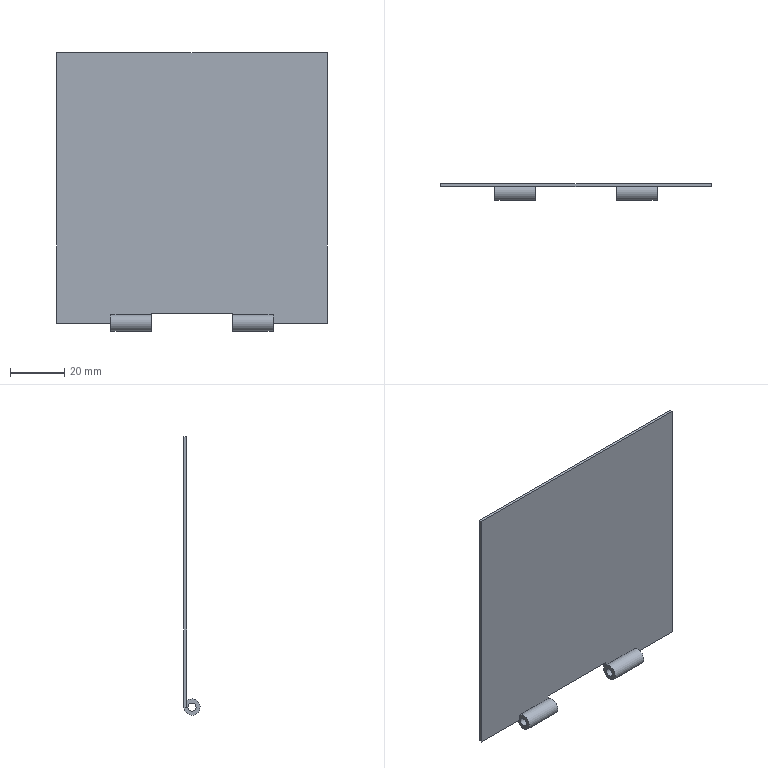Component | NX | PART_7 | 1 solid | 16 faces | box 100 x 6 x 103 mm | volume 10485 mm3 | plane 12 | cylinder 4 | commonest cylinder face diameters 6 x2 3 x2
STEP:
#1=CARTESIAN_POINT('',(0.,0.,0.));
#2=DIRECTION('',(0.,0.,1.));
#3=DIRECTION('',(1.,0.,0.));
#4=AXIS2_PLACEMENT_3D('',#1,#2,#3);
#5=CARTESIAN_POINT('',(-30.,28.,-0.));
#6=VERTEX_POINT('',#5);
#7=CARTESIAN_POINT('',(-30.,29.,-0.));
#8=VERTEX_POINT('',#7);
#9=CARTESIAN_POINT('',(-30.,29.,-0.));
#10=DIRECTION('',(0.,1.,0.));
#11=VECTOR('',#10,1.);
#12=LINE('',#9,#11);
#13=CARTESIAN_POINT('',(50.,29.,-0.));
#14=DIRECTION('',(0.,-0.,1.));
#15=DIRECTION('',(0.,-1.,-0.));
#16=AXIS2_PLACEMENT_3D('',#13,#14,#15);
#17=PLANE('',#16);
#18=CARTESIAN_POINT('',(0.,-80.));
#19=DIRECTION('',(-1.,0.));
#20=VECTOR('',#19,1.);
#21=LINE('',#18,#20);
#22=(GEOMETRIC_REPRESENTATION_CONTEXT(2)PARAMETRIC_REPRESENTATION_CONTEXT()REPRESENTATION_CONTEXT('',''));
#23=DEFINITIONAL_REPRESENTATION('',(#21),#22);
#24=PCURVE('',#17,#23);
#25=CARTESIAN_POINT('',(-30.,26.,-0.));
#26=DIRECTION('',(1.,0.,0.));
#27=DIRECTION('',(0.,0.,1.));
#28=AXIS2_PLACEMENT_3D('',#25,#26,#27);
#29=PLANE('',#28);
#30=CARTESIAN_POINT('',(0.,-3.));
#31=DIRECTION('',(0.,-1.));
#32=VECTOR('',#31,1.);
#33=LINE('',#30,#32);
#34=(GEOMETRIC_REPRESENTATION_CONTEXT(2)PARAMETRIC_REPRESENTATION_CONTEXT()REPRESENTATION_CONTEXT('',''));
#35=DEFINITIONAL_REPRESENTATION('',(#33),#34);
#36=PCURVE('',#29,#35);
#37=SURFACE_CURVE('',#12,(#24,#36),.PCURVE_S1.);
#38=EDGE_CURVE('',#6,#8,#37,.T.);
#39=ORIENTED_EDGE('',*,*,#38,.F.);
#40=CARTESIAN_POINT('',(-50.,28.,-0.));
#41=VERTEX_POINT('',#40);
#42=CARTESIAN_POINT('',(50.,28.,-0.));
#43=DIRECTION('',(-1.,0.,0.));
#44=VECTOR('',#43,1.);
#45=LINE('',#42,#44);
#46=CARTESIAN_POINT('',(1.,0.));
#47=DIRECTION('',(0.,-1.));
#48=VECTOR('',#47,1.);
#49=LINE('',#46,#48);
#50=(GEOMETRIC_REPRESENTATION_CONTEXT(2)PARAMETRIC_REPRESENTATION_CONTEXT()REPRESENTATION_CONTEXT('',''));
#51=DEFINITIONAL_REPRESENTATION('',(#49),#50);
#52=PCURVE('',#17,#51);
#53=CARTESIAN_POINT('',(50.,28.,100.));
#54=DIRECTION('',(0.,1.,0.));
#55=DIRECTION('',(0.,-0.,1.));
#56=AXIS2_PLACEMENT_3D('',#53,#54,#55);
#57=PLANE('',#56);
#58=CARTESIAN_POINT('',(-100.,0.));
#59=DIRECTION('',(0.,-1.));
#60=VECTOR('',#59,1.);
#61=LINE('',#58,#60);
#62=(GEOMETRIC_REPRESENTATION_CONTEXT(2)PARAMETRIC_REPRESENTATION_CONTEXT()REPRESENTATION_CONTEXT('',''));
#63=DEFINITIONAL_REPRESENTATION('',(#61),#62);
#64=PCURVE('',#57,#63);
#65=SURFACE_CURVE('',#45,(#52,#64),.PCURVE_S1.);
#66=EDGE_CURVE('',#6,#41,#65,.T.);
#67=ORIENTED_EDGE('',*,*,#66,.T.);
#68=CARTESIAN_POINT('',(-50.,29.,-0.));
#69=VERTEX_POINT('',#68);
#70=CARTESIAN_POINT('',(-50.,31.,-0.));
#71=DIRECTION('',(0.,1.,0.));
#72=VECTOR('',#71,1.);
#73=LINE('',#70,#72);
#74=CARTESIAN_POINT('',(-2.,-100.));
#75=DIRECTION('',(-1.,0.));
#76=VECTOR('',#75,1.);
#77=LINE('',#74,#76);
#78=(GEOMETRIC_REPRESENTATION_CONTEXT(2)PARAMETRIC_REPRESENTATION_CONTEXT()REPRESENTATION_CONTEXT('',''));
#79=DEFINITIONAL_REPRESENTATION('',(#77),#78);
#80=PCURVE('',#17,#79);
#81=CARTESIAN_POINT('',(-50.,31.,100.));
#82=DIRECTION('',(-1.,0.,0.));
#83=DIRECTION('',(0.,0.,-1.));
#84=AXIS2_PLACEMENT_3D('',#81,#82,#83);
#85=PLANE('',#84);
#86=CARTESIAN_POINT('',(100.,0.));
#87=DIRECTION('',(-0.,-1.));
#88=VECTOR('',#87,1.);
#89=LINE('',#86,#88);
#90=(GEOMETRIC_REPRESENTATION_CONTEXT(2)PARAMETRIC_REPRESENTATION_CONTEXT()REPRESENTATION_CONTEXT('',''));
#91=DEFINITIONAL_REPRESENTATION('',(#89),#90);
#92=PCURVE('',#85,#91);
#93=SURFACE_CURVE('',#73,(#80,#92),.PCURVE_S1.);
#94=EDGE_CURVE('',#41,#69,#93,.T.);
#95=ORIENTED_EDGE('',*,*,#94,.T.);
#96=CARTESIAN_POINT('',(50.,29.,-0.));
#97=DIRECTION('',(-1.,0.,0.));
#98=VECTOR('',#97,1.);
#99=LINE('',#96,#98);
#100=CARTESIAN_POINT('',(0.,0.));
#101=DIRECTION('',(0.,-1.));
#102=VECTOR('',#101,1.);
#103=LINE('',#100,#102);
#104=(GEOMETRIC_REPRESENTATION_CONTEXT(2)PARAMETRIC_REPRESENTATION_CONTEXT()REPRESENTATION_CONTEXT('',''));
#105=DEFINITIONAL_REPRESENTATION('',(#103),#104);
#106=PCURVE('',#17,#105);
#107=CARTESIAN_POINT('',(50.,29.,-0.));
#108=DIRECTION('',(0.,-1.,-0.));
#109=DIRECTION('',(0.,0.,-1.));
#110=AXIS2_PLACEMENT_3D('',#107,#108,#109);
#111=PLANE('',#110);
#112=CARTESIAN_POINT('',(-0.,0.));
#113=DIRECTION('',(0.,-1.));
#114=VECTOR('',#113,1.);
#115=LINE('',#112,#114);
#116=(GEOMETRIC_REPRESENTATION_CONTEXT(2)PARAMETRIC_REPRESENTATION_CONTEXT()REPRESENTATION_CONTEXT('',''));
#117=DEFINITIONAL_REPRESENTATION('',(#115),#116);
#118=PCURVE('',#111,#117);
#119=SURFACE_CURVE('',#99,(#106,#118),.PCURVE_S1.);
#120=EDGE_CURVE('',#8,#69,#119,.T.);
#121=ORIENTED_EDGE('',*,*,#120,.F.);
#122=EDGE_LOOP('',(#39,#67,#95,#121));
#123=FACE_BOUND('',#122,.T.);
#124=ADVANCED_FACE('',(#123),#17,.F.);
#125=CARTESIAN_POINT('',(-30.,28.,2.236));
#126=VERTEX_POINT('',#125);
#127=CARTESIAN_POINT('',(-15.,28.,2.236));
#128=VERTEX_POINT('',#127);
#129=CARTESIAN_POINT('',(-30.,28.,2.236));
#130=DIRECTION('',(1.,0.,0.));
#131=VECTOR('',#130,1.);
#132=LINE('',#129,#131);
#133=CARTESIAN_POINT('',(-97.764,-80.));
#134=DIRECTION('',(0.,1.));
#135=VECTOR('',#134,1.);
#136=LINE('',#133,#135);
#137=(GEOMETRIC_REPRESENTATION_CONTEXT(2)PARAMETRIC_REPRESENTATION_CONTEXT()REPRESENTATION_CONTEXT('',''));
#138=DEFINITIONAL_REPRESENTATION('',(#136),#137);
#139=PCURVE('',#57,#138);
#140=CARTESIAN_POINT('',(-30.,26.,-0.));
#141=DIRECTION('',(1.,0.,0.));
#142=DIRECTION('',(0.,0.,1.));
#143=AXIS2_PLACEMENT_3D('',#140,#141,#142);
#144=CYLINDRICAL_SURFACE('',#143,3.);
#145=CARTESIAN_POINT('',(-0.7297,0.));
#146=DIRECTION('',(0.,1.));
#147=VECTOR('',#146,1.);
#148=LINE('',#145,#147);
#149=(GEOMETRIC_REPRESENTATION_CONTEXT(2)PARAMETRIC_REPRESENTATION_CONTEXT()REPRESENTATION_CONTEXT('',''));
#150=DEFINITIONAL_REPRESENTATION('',(#148),#149);
#151=PCURVE('',#144,#150);
#152=SURFACE_CURVE('',#132,(#139,#151),.PCURVE_S1.);
#153=EDGE_CURVE('',#126,#128,#152,.T.);
#154=ORIENTED_EDGE('',*,*,#153,.T.);
#155=CARTESIAN_POINT('',(-15.,28.,3.5));
#156=VERTEX_POINT('',#155);
#157=CARTESIAN_POINT('',(-15.,28.,100.));
#158=DIRECTION('',(0.,-0.,1.));
#159=VECTOR('',#158,1.);
#160=LINE('',#157,#159);
#161=CARTESIAN_POINT('',(0.,-65.));
#162=DIRECTION('',(1.,0.));
#163=VECTOR('',#162,1.);
#164=LINE('',#161,#163);
#165=(GEOMETRIC_REPRESENTATION_CONTEXT(2)PARAMETRIC_REPRESENTATION_CONTEXT()REPRESENTATION_CONTEXT('',''));
#166=DEFINITIONAL_REPRESENTATION('',(#164),#165);
#167=PCURVE('',#57,#166);
#168=CARTESIAN_POINT('',(-15.,26.,-0.));
#169=DIRECTION('',(1.,0.,0.));
#170=DIRECTION('',(0.,0.,1.));
#171=AXIS2_PLACEMENT_3D('',#168,#169,#170);
#172=PLANE('',#171);
#173=CARTESIAN_POINT('',(100.,-2.));
#174=DIRECTION('',(1.,0.));
#175=VECTOR('',#174,1.);
#176=LINE('',#173,#175);
#177=(GEOMETRIC_REPRESENTATION_CONTEXT(2)PARAMETRIC_REPRESENTATION_CONTEXT()REPRESENTATION_CONTEXT('',''));
#178=DEFINITIONAL_REPRESENTATION('',(#176),#177);
#179=PCURVE('',#172,#178);
#180=SURFACE_CURVE('',#160,(#167,#179),.PCURVE_S1.);
#181=EDGE_CURVE('',#128,#156,#180,.T.);
#182=ORIENTED_EDGE('',*,*,#181,.T.);
#183=CARTESIAN_POINT('',(15.,28.,3.5));
#184=VERTEX_POINT('',#183);
#185=CARTESIAN_POINT('',(50.,28.,3.5));
#186=DIRECTION('',(1.,0.,0.));
#187=VECTOR('',#186,1.);
#188=LINE('',#185,#187);
#189=CARTESIAN_POINT('',(-96.5,0.));
#190=DIRECTION('',(0.,1.));
#191=VECTOR('',#190,1.);
#192=LINE('',#189,#191);
#193=(GEOMETRIC_REPRESENTATION_CONTEXT(2)PARAMETRIC_REPRESENTATION_CONTEXT()REPRESENTATION_CONTEXT('',''));
#194=DEFINITIONAL_REPRESENTATION('',(#192),#193);
#195=PCURVE('',#57,#194);
#196=CARTESIAN_POINT('',(0.,28.5,3.5));
#197=DIRECTION('',(0.,0.,1.));
#198=DIRECTION('',(-1.,0.,0.));
#199=AXIS2_PLACEMENT_3D('',#196,#197,#198);
#200=PLANE('',#199);
#201=CARTESIAN_POINT('',(-50.,0.5));
#202=DIRECTION('',(-1.,0.));
#203=VECTOR('',#202,1.);
#204=LINE('',#201,#203);
#205=(GEOMETRIC_REPRESENTATION_CONTEXT(2)PARAMETRIC_REPRESENTATION_CONTEXT()REPRESENTATION_CONTEXT('',''));
#206=DEFINITIONAL_REPRESENTATION('',(#204),#205);
#207=PCURVE('',#200,#206);
#208=SURFACE_CURVE('',#188,(#195,#207),.PCURVE_S1.);
#209=EDGE_CURVE('',#156,#184,#208,.T.);
#210=ORIENTED_EDGE('',*,*,#209,.T.);
#211=CARTESIAN_POINT('',(15.,28.,2.236));
#212=VERTEX_POINT('',#211);
#213=CARTESIAN_POINT('',(15.,28.,100.));
#214=DIRECTION('',(0.,-0.,1.));
#215=VECTOR('',#214,1.);
#216=LINE('',#213,#215);
#217=CARTESIAN_POINT('',(0.,-35.));
#218=DIRECTION('',(1.,0.));
#219=VECTOR('',#218,1.);
#220=LINE('',#217,#219);
#221=(GEOMETRIC_REPRESENTATION_CONTEXT(2)PARAMETRIC_REPRESENTATION_CONTEXT()REPRESENTATION_CONTEXT('',''));
#222=DEFINITIONAL_REPRESENTATION('',(#220),#221);
#223=PCURVE('',#57,#222);
#224=CARTESIAN_POINT('',(15.,26.,-0.));
#225=DIRECTION('',(1.,0.,0.));
#226=DIRECTION('',(0.,0.,1.));
#227=AXIS2_PLACEMENT_3D('',#224,#225,#226);
#228=PLANE('',#227);
#229=CARTESIAN_POINT('',(100.,-2.));
#230=DIRECTION('',(1.,0.));
#231=VECTOR('',#230,1.);
#232=LINE('',#229,#231);
#233=(GEOMETRIC_REPRESENTATION_CONTEXT(2)PARAMETRIC_REPRESENTATION_CONTEXT()REPRESENTATION_CONTEXT('',''));
#234=DEFINITIONAL_REPRESENTATION('',(#232),#233);
#235=PCURVE('',#228,#234);
#236=SURFACE_CURVE('',#216,(#223,#235),.PCURVE_S1.);
#237=EDGE_CURVE('',#212,#184,#236,.T.);
#238=ORIENTED_EDGE('',*,*,#237,.F.);
#239=CARTESIAN_POINT('',(30.,28.,2.236));
#240=VERTEX_POINT('',#239);
#241=CARTESIAN_POINT('',(30.,28.,2.236));
#242=DIRECTION('',(-1.,0.,0.));
#243=VECTOR('',#242,1.);
#244=LINE('',#241,#243);
#245=CARTESIAN_POINT('',(-97.764,-20.));
#246=DIRECTION('',(0.,-1.));
#247=VECTOR('',#246,1.);
#248=LINE('',#245,#247);
#249=(GEOMETRIC_REPRESENTATION_CONTEXT(2)PARAMETRIC_REPRESENTATION_CONTEXT()REPRESENTATION_CONTEXT('',''));
#250=DEFINITIONAL_REPRESENTATION('',(#248),#249);
#251=PCURVE('',#57,#250);
#252=CARTESIAN_POINT('',(30.,26.,-0.));
#253=DIRECTION('',(-1.,0.,0.));
#254=DIRECTION('',(0.,0.,-1.));
#255=AXIS2_PLACEMENT_3D('',#252,#253,#254);
#256=CYLINDRICAL_SURFACE('',#255,3.);
#257=CARTESIAN_POINT('',(3.871,0.));
#258=DIRECTION('',(0.,1.));
#259=VECTOR('',#258,1.);
#260=LINE('',#257,#259);
#261=(GEOMETRIC_REPRESENTATION_CONTEXT(2)PARAMETRIC_REPRESENTATION_CONTEXT()REPRESENTATION_CONTEXT('',''));
#262=DEFINITIONAL_REPRESENTATION('',(#260),#261);
#263=PCURVE('',#256,#262);
#264=SURFACE_CURVE('',#244,(#251,#263),.PCURVE_S1.);
#265=EDGE_CURVE('',#240,#212,#264,.T.);
#266=ORIENTED_EDGE('',*,*,#265,.F.);
#267=CARTESIAN_POINT('',(30.,28.,-0.));
#268=VERTEX_POINT('',#267);
#269=CARTESIAN_POINT('',(30.,28.,100.));
#270=DIRECTION('',(0.,0.,-1.));
#271=VECTOR('',#270,1.);
#272=LINE('',#269,#271);
#273=CARTESIAN_POINT('',(0.,-20.));
#274=DIRECTION('',(-1.,0.));
#275=VECTOR('',#274,1.);
#276=LINE('',#273,#275);
#277=(GEOMETRIC_REPRESENTATION_CONTEXT(2)PARAMETRIC_REPRESENTATION_CONTEXT()REPRESENTATION_CONTEXT('',''));
#278=DEFINITIONAL_REPRESENTATION('',(#276),#277);
#279=PCURVE('',#57,#278);
#280=CARTESIAN_POINT('',(30.,26.,-0.));
#281=DIRECTION('',(1.,0.,0.));
#282=DIRECTION('',(0.,0.,1.));
#283=AXIS2_PLACEMENT_3D('',#280,#281,#282);
#284=PLANE('',#283);
#285=CARTESIAN_POINT('',(100.,-2.));
#286=DIRECTION('',(-1.,-0.));
#287=VECTOR('',#286,1.);
#288=LINE('',#285,#287);
#289=(GEOMETRIC_REPRESENTATION_CONTEXT(2)PARAMETRIC_REPRESENTATION_CONTEXT()REPRESENTATION_CONTEXT('',''));
#290=DEFINITIONAL_REPRESENTATION('',(#288),#289);
#291=PCURVE('',#284,#290);
#292=SURFACE_CURVE('',#272,(#279,#291),.PCURVE_S1.);
#293=EDGE_CURVE('',#240,#268,#292,.T.);
#294=ORIENTED_EDGE('',*,*,#293,.T.);
#295=CARTESIAN_POINT('',(50.,28.,-0.));
#296=VERTEX_POINT('',#295);
#297=CARTESIAN_POINT('',(50.,28.,-0.));
#298=DIRECTION('',(-1.,0.,0.));
#299=VECTOR('',#298,1.);
#300=LINE('',#297,#299);
#301=CARTESIAN_POINT('',(-100.,0.));
#302=DIRECTION('',(0.,-1.));
#303=VECTOR('',#302,1.);
#304=LINE('',#301,#303);
#305=(GEOMETRIC_REPRESENTATION_CONTEXT(2)PARAMETRIC_REPRESENTATION_CONTEXT()REPRESENTATION_CONTEXT('',''));
#306=DEFINITIONAL_REPRESENTATION('',(#304),#305);
#307=PCURVE('',#57,#306);
#308=CARTESIAN_POINT('',(50.,29.,-0.));
#309=DIRECTION('',(0.,-0.,1.));
#310=DIRECTION('',(0.,-1.,-0.));
#311=AXIS2_PLACEMENT_3D('',#308,#309,#310);
#312=PLANE('',#311);
#313=CARTESIAN_POINT('',(1.,0.));
#314=DIRECTION('',(0.,-1.));
#315=VECTOR('',#314,1.);
#316=LINE('',#313,#315);
#317=(GEOMETRIC_REPRESENTATION_CONTEXT(2)PARAMETRIC_REPRESENTATION_CONTEXT()REPRESENTATION_CONTEXT('',''));
#318=DEFINITIONAL_REPRESENTATION('',(#316),#317);
#319=PCURVE('',#312,#318);
#320=SURFACE_CURVE('',#300,(#307,#319),.PCURVE_S1.);
#321=EDGE_CURVE('',#296,#268,#320,.T.);
#322=ORIENTED_EDGE('',*,*,#321,.F.);
#323=CARTESIAN_POINT('',(50.,28.,100.));
#324=VERTEX_POINT('',#323);
#325=CARTESIAN_POINT('',(50.,28.,100.));
#326=DIRECTION('',(0.,0.,-1.));
#327=VECTOR('',#326,1.);
#328=LINE('',#325,#327);
#329=CARTESIAN_POINT('',(0.,0.));
#330=DIRECTION('',(-1.,0.));
#331=VECTOR('',#330,1.);
#332=LINE('',#329,#331);
#333=(GEOMETRIC_REPRESENTATION_CONTEXT(2)PARAMETRIC_REPRESENTATION_CONTEXT()REPRESENTATION_CONTEXT('',''));
#334=DEFINITIONAL_REPRESENTATION('',(#332),#333);
#335=PCURVE('',#57,#334);
#336=CARTESIAN_POINT('',(50.,31.,100.));
#337=DIRECTION('',(-1.,0.,0.));
#338=DIRECTION('',(0.,0.,-1.));
#339=AXIS2_PLACEMENT_3D('',#336,#337,#338);
#340=PLANE('',#339);
#341=CARTESIAN_POINT('',(0.,3.));
#342=DIRECTION('',(1.,-0.));
#343=VECTOR('',#342,1.);
#344=LINE('',#341,#343);
#345=(GEOMETRIC_REPRESENTATION_CONTEXT(2)PARAMETRIC_REPRESENTATION_CONTEXT()REPRESENTATION_CONTEXT('',''));
#346=DEFINITIONAL_REPRESENTATION('',(#344),#345);
#347=PCURVE('',#340,#346);
#348=SURFACE_CURVE('',#328,(#335,#347),.PCURVE_S1.);
#349=EDGE_CURVE('',#324,#296,#348,.T.);
#350=ORIENTED_EDGE('',*,*,#349,.F.);
#351=CARTESIAN_POINT('',(-50.,28.,100.));
#352=VERTEX_POINT('',#351);
#353=CARTESIAN_POINT('',(50.,28.,100.));
#354=DIRECTION('',(-1.,0.,0.));
#355=VECTOR('',#354,1.);
#356=LINE('',#353,#355);
#357=CARTESIAN_POINT('',(0.,0.));
#358=DIRECTION('',(0.,-1.));
#359=VECTOR('',#358,1.);
#360=LINE('',#357,#359);
#361=(GEOMETRIC_REPRESENTATION_CONTEXT(2)PARAMETRIC_REPRESENTATION_CONTEXT()REPRESENTATION_CONTEXT('',''));
#362=DEFINITIONAL_REPRESENTATION('',(#360),#361);
#363=PCURVE('',#57,#362);
#364=CARTESIAN_POINT('',(0.,31.,100.));
#365=DIRECTION('',(0.,0.,-1.));
#366=DIRECTION('',(0.,-1.,0.));
#367=AXIS2_PLACEMENT_3D('',#364,#365,#366);
#368=PLANE('',#367);
#369=CARTESIAN_POINT('',(3.,-50.));
#370=DIRECTION('',(0.,1.));
#371=VECTOR('',#370,1.);
#372=LINE('',#369,#371);
#373=(GEOMETRIC_REPRESENTATION_CONTEXT(2)PARAMETRIC_REPRESENTATION_CONTEXT()REPRESENTATION_CONTEXT('',''));
#374=DEFINITIONAL_REPRESENTATION('',(#372),#373);
#375=PCURVE('',#368,#374);
#376=SURFACE_CURVE('',#356,(#363,#375),.PCURVE_S1.);
#377=EDGE_CURVE('',#324,#352,#376,.T.);
#378=ORIENTED_EDGE('',*,*,#377,.T.);
#379=CARTESIAN_POINT('',(-50.,28.,100.));
#380=DIRECTION('',(0.,0.,-1.));
#381=VECTOR('',#380,1.);
#382=LINE('',#379,#381);
#383=CARTESIAN_POINT('',(0.,-100.));
#384=DIRECTION('',(-1.,0.));
#385=VECTOR('',#384,1.);
#386=LINE('',#383,#385);
#387=(GEOMETRIC_REPRESENTATION_CONTEXT(2)PARAMETRIC_REPRESENTATION_CONTEXT()REPRESENTATION_CONTEXT('',''));
#388=DEFINITIONAL_REPRESENTATION('',(#386),#387);
#389=PCURVE('',#57,#388);
#390=CARTESIAN_POINT('',(0.,3.));
#391=DIRECTION('',(1.,-0.));
#392=VECTOR('',#391,1.);
#393=LINE('',#390,#392);
#394=(GEOMETRIC_REPRESENTATION_CONTEXT(2)PARAMETRIC_REPRESENTATION_CONTEXT()REPRESENTATION_CONTEXT('',''));
#395=DEFINITIONAL_REPRESENTATION('',(#393),#394);
#396=PCURVE('',#85,#395);
#397=SURFACE_CURVE('',#382,(#389,#396),.PCURVE_S1.);
#398=EDGE_CURVE('',#352,#41,#397,.T.);
#399=ORIENTED_EDGE('',*,*,#398,.T.);
#400=ORIENTED_EDGE('',*,*,#66,.F.);
#401=CARTESIAN_POINT('',(-30.,28.,100.));
#402=DIRECTION('',(0.,0.,-1.));
#403=VECTOR('',#402,1.);
#404=LINE('',#401,#403);
#405=CARTESIAN_POINT('',(0.,-80.));
#406=DIRECTION('',(-1.,0.));
#407=VECTOR('',#406,1.);
#408=LINE('',#405,#407);
#409=(GEOMETRIC_REPRESENTATION_CONTEXT(2)PARAMETRIC_REPRESENTATION_CONTEXT()REPRESENTATION_CONTEXT('',''));
#410=DEFINITIONAL_REPRESENTATION('',(#408),#409);
#411=PCURVE('',#57,#410);
#412=CARTESIAN_POINT('',(100.,-2.));
#413=DIRECTION('',(-1.,-0.));
#414=VECTOR('',#413,1.);
#415=LINE('',#412,#414);
#416=(GEOMETRIC_REPRESENTATION_CONTEXT(2)PARAMETRIC_REPRESENTATION_CONTEXT()REPRESENTATION_CONTEXT('',''));
#417=DEFINITIONAL_REPRESENTATION('',(#415),#416);
#418=PCURVE('',#29,#417);
#419=SURFACE_CURVE('',#404,(#411,#418),.PCURVE_S1.);
#420=EDGE_CURVE('',#126,#6,#419,.T.);
#421=ORIENTED_EDGE('',*,*,#420,.F.);
#422=EDGE_LOOP('',(#154,#182,#210,#238,#266,#294,#322,#350,#378,#399,#400,#421));
#423=FACE_BOUND('',#422,.T.);
#424=ADVANCED_FACE('',(#423),#57,.F.);
#425=CARTESIAN_POINT('',(15.,29.,3.5));
#426=VERTEX_POINT('',#425);
#427=CARTESIAN_POINT('',(-15.,29.,3.5));
#428=VERTEX_POINT('',#427);
#429=CARTESIAN_POINT('',(50.,29.,3.5));
#430=DIRECTION('',(-1.,0.,0.));
#431=VECTOR('',#430,1.);
#432=LINE('',#429,#431);
#433=CARTESIAN_POINT('',(-3.5,0.));
#434=DIRECTION('',(0.,-1.));
#435=VECTOR('',#434,1.);
#436=LINE('',#433,#435);
#437=(GEOMETRIC_REPRESENTATION_CONTEXT(2)PARAMETRIC_REPRESENTATION_CONTEXT()REPRESENTATION_CONTEXT('',''));
#438=DEFINITIONAL_REPRESENTATION('',(#436),#437);
#439=PCURVE('',#111,#438);
#440=CARTESIAN_POINT('',(-50.,-0.5));
#441=DIRECTION('',(1.,0.));
#442=VECTOR('',#441,1.);
#443=LINE('',#440,#442);
#444=(GEOMETRIC_REPRESENTATION_CONTEXT(2)PARAMETRIC_REPRESENTATION_CONTEXT()REPRESENTATION_CONTEXT('',''));
#445=DEFINITIONAL_REPRESENTATION('',(#443),#444);
#446=PCURVE('',#200,#445);
#447=SURFACE_CURVE('',#432,(#439,#446),.PCURVE_S1.);
#448=EDGE_CURVE('',#426,#428,#447,.T.);
#449=ORIENTED_EDGE('',*,*,#448,.T.);
#450=CARTESIAN_POINT('',(-15.,29.,-0.));
#451=VERTEX_POINT('',#450);
#452=CARTESIAN_POINT('',(-15.,29.,-0.));
#453=DIRECTION('',(0.,0.,-1.));
#454=VECTOR('',#453,1.);
#455=LINE('',#452,#454);
#456=CARTESIAN_POINT('',(0.,-65.));
#457=DIRECTION('',(1.,0.));
#458=VECTOR('',#457,1.);
#459=LINE('',#456,#458);
#460=(GEOMETRIC_REPRESENTATION_CONTEXT(2)PARAMETRIC_REPRESENTATION_CONTEXT()REPRESENTATION_CONTEXT('',''));
#461=DEFINITIONAL_REPRESENTATION('',(#459),#460);
#462=PCURVE('',#111,#461);
#463=CARTESIAN_POINT('',(0.,-3.));
#464=DIRECTION('',(-1.,-0.));
#465=VECTOR('',#464,1.);
#466=LINE('',#463,#465);
#467=(GEOMETRIC_REPRESENTATION_CONTEXT(2)PARAMETRIC_REPRESENTATION_CONTEXT()REPRESENTATION_CONTEXT('',''));
#468=DEFINITIONAL_REPRESENTATION('',(#466),#467);
#469=PCURVE('',#172,#468);
#470=SURFACE_CURVE('',#455,(#462,#469),.PCURVE_S1.);
#471=EDGE_CURVE('',#428,#451,#470,.T.);
#472=ORIENTED_EDGE('',*,*,#471,.T.);
#473=CARTESIAN_POINT('',(-30.,29.,-0.));
#474=DIRECTION('',(1.,0.,0.));
#475=VECTOR('',#474,1.);
#476=LINE('',#473,#475);
#477=CARTESIAN_POINT('',(-0.,-80.));
#478=DIRECTION('',(0.,1.));
#479=VECTOR('',#478,1.);
#480=LINE('',#477,#479);
#481=(GEOMETRIC_REPRESENTATION_CONTEXT(2)PARAMETRIC_REPRESENTATION_CONTEXT()REPRESENTATION_CONTEXT('',''));
#482=DEFINITIONAL_REPRESENTATION('',(#480),#481);
#483=PCURVE('',#111,#482);
#484=CARTESIAN_POINT('',(4.712,0.));
#485=DIRECTION('',(0.,1.));
#486=VECTOR('',#485,1.);
#487=LINE('',#484,#486);
#488=(GEOMETRIC_REPRESENTATION_CONTEXT(2)PARAMETRIC_REPRESENTATION_CONTEXT()REPRESENTATION_CONTEXT('',''));
#489=DEFINITIONAL_REPRESENTATION('',(#487),#488);
#490=PCURVE('',#144,#489);
#491=SURFACE_CURVE('',#476,(#483,#490),.PCURVE_S1.);
#492=EDGE_CURVE('',#8,#451,#491,.T.);
#493=ORIENTED_EDGE('',*,*,#492,.F.);
#494=ORIENTED_EDGE('',*,*,#120,.T.);
#495=CARTESIAN_POINT('',(-50.,29.,100.));
#496=VERTEX_POINT('',#495);
#497=CARTESIAN_POINT('',(-50.,29.,-0.));
#498=DIRECTION('',(0.,-0.,1.));
#499=VECTOR('',#498,1.);
#500=LINE('',#497,#499);
#501=CARTESIAN_POINT('',(0.,-100.));
#502=DIRECTION('',(-1.,0.));
#503=VECTOR('',#502,1.);
#504=LINE('',#501,#503);
#505=(GEOMETRIC_REPRESENTATION_CONTEXT(2)PARAMETRIC_REPRESENTATION_CONTEXT()REPRESENTATION_CONTEXT('',''));
#506=DEFINITIONAL_REPRESENTATION('',(#504),#505);
#507=PCURVE('',#111,#506);
#508=CARTESIAN_POINT('',(100.,2.));
#509=DIRECTION('',(-1.,0.));
#510=VECTOR('',#509,1.);
#511=LINE('',#508,#510);
#512=(GEOMETRIC_REPRESENTATION_CONTEXT(2)PARAMETRIC_REPRESENTATION_CONTEXT()REPRESENTATION_CONTEXT('',''));
#513=DEFINITIONAL_REPRESENTATION('',(#511),#512);
#514=PCURVE('',#85,#513);
#515=SURFACE_CURVE('',#500,(#507,#514),.PCURVE_S1.);
#516=EDGE_CURVE('',#69,#496,#515,.T.);
#517=ORIENTED_EDGE('',*,*,#516,.T.);
#518=CARTESIAN_POINT('',(50.,29.,100.));
#519=VERTEX_POINT('',#518);
#520=CARTESIAN_POINT('',(0.,29.,100.));
#521=DIRECTION('',(-1.,0.,0.));
#522=VECTOR('',#521,1.);
#523=LINE('',#520,#522);
#524=CARTESIAN_POINT('',(-100.,-50.));
#525=DIRECTION('',(0.,-1.));
#526=VECTOR('',#525,1.);
#527=LINE('',#524,#526);
#528=(GEOMETRIC_REPRESENTATION_CONTEXT(2)PARAMETRIC_REPRESENTATION_CONTEXT()REPRESENTATION_CONTEXT('',''));
#529=DEFINITIONAL_REPRESENTATION('',(#527),#528);
#530=PCURVE('',#111,#529);
#531=CARTESIAN_POINT('',(2.,0.));
#532=DIRECTION('',(0.,1.));
#533=VECTOR('',#532,1.);
#534=LINE('',#531,#533);
#535=(GEOMETRIC_REPRESENTATION_CONTEXT(2)PARAMETRIC_REPRESENTATION_CONTEXT()REPRESENTATION_CONTEXT('',''));
#536=DEFINITIONAL_REPRESENTATION('',(#534),#535);
#537=PCURVE('',#368,#536);
#538=SURFACE_CURVE('',#523,(#530,#537),.PCURVE_S1.);
#539=EDGE_CURVE('',#519,#496,#538,.T.);
#540=ORIENTED_EDGE('',*,*,#539,.F.);
#541=CARTESIAN_POINT('',(50.,29.,-0.));
#542=VERTEX_POINT('',#541);
#543=CARTESIAN_POINT('',(50.,29.,-0.));
#544=DIRECTION('',(0.,-0.,1.));
#545=VECTOR('',#544,1.);
#546=LINE('',#543,#545);
#547=CARTESIAN_POINT('',(0.,0.));
#548=DIRECTION('',(-1.,0.));
#549=VECTOR('',#548,1.);
#550=LINE('',#547,#549);
#551=(GEOMETRIC_REPRESENTATION_CONTEXT(2)PARAMETRIC_REPRESENTATION_CONTEXT()REPRESENTATION_CONTEXT('',''));
#552=DEFINITIONAL_REPRESENTATION('',(#550),#551);
#553=PCURVE('',#111,#552);
#554=CARTESIAN_POINT('',(100.,2.));
#555=DIRECTION('',(-1.,0.));
#556=VECTOR('',#555,1.);
#557=LINE('',#554,#556);
#558=(GEOMETRIC_REPRESENTATION_CONTEXT(2)PARAMETRIC_REPRESENTATION_CONTEXT()REPRESENTATION_CONTEXT('',''));
#559=DEFINITIONAL_REPRESENTATION('',(#557),#558);
#560=PCURVE('',#340,#559);
#561=SURFACE_CURVE('',#546,(#553,#560),.PCURVE_S1.);
#562=EDGE_CURVE('',#542,#519,#561,.T.);
#563=ORIENTED_EDGE('',*,*,#562,.F.);
#564=CARTESIAN_POINT('',(30.,29.,-0.));
#565=VERTEX_POINT('',#564);
#566=CARTESIAN_POINT('',(50.,29.,-0.));
#567=DIRECTION('',(-1.,0.,0.));
#568=VECTOR('',#567,1.);
#569=LINE('',#566,#568);
#570=CARTESIAN_POINT('',(-0.,0.));
#571=DIRECTION('',(0.,-1.));
#572=VECTOR('',#571,1.);
#573=LINE('',#570,#572);
#574=(GEOMETRIC_REPRESENTATION_CONTEXT(2)PARAMETRIC_REPRESENTATION_CONTEXT()REPRESENTATION_CONTEXT('',''));
#575=DEFINITIONAL_REPRESENTATION('',(#573),#574);
#576=PCURVE('',#111,#575);
#577=CARTESIAN_POINT('',(0.,0.));
#578=DIRECTION('',(0.,-1.));
#579=VECTOR('',#578,1.);
#580=LINE('',#577,#579);
#581=(GEOMETRIC_REPRESENTATION_CONTEXT(2)PARAMETRIC_REPRESENTATION_CONTEXT()REPRESENTATION_CONTEXT('',''));
#582=DEFINITIONAL_REPRESENTATION('',(#580),#581);
#583=PCURVE('',#312,#582);
#584=SURFACE_CURVE('',#569,(#576,#583),.PCURVE_S1.);
#585=EDGE_CURVE('',#542,#565,#584,.T.);
#586=ORIENTED_EDGE('',*,*,#585,.T.);
#587=CARTESIAN_POINT('',(15.,29.,-0.));
#588=VERTEX_POINT('',#587);
#589=CARTESIAN_POINT('',(50.,29.,-0.));
#590=DIRECTION('',(-1.,0.,0.));
#591=VECTOR('',#590,1.);
#592=LINE('',#589,#591);
#593=CARTESIAN_POINT('',(-0.,0.));
#594=DIRECTION('',(0.,-1.));
#595=VECTOR('',#594,1.);
#596=LINE('',#593,#595);
#597=(GEOMETRIC_REPRESENTATION_CONTEXT(2)PARAMETRIC_REPRESENTATION_CONTEXT()REPRESENTATION_CONTEXT('',''));
#598=DEFINITIONAL_REPRESENTATION('',(#596),#597);
#599=PCURVE('',#111,#598);
#600=CARTESIAN_POINT('',(-1.571,-20.));
#601=DIRECTION('',(0.,1.));
#602=VECTOR('',#601,1.);
#603=LINE('',#600,#602);
#604=(GEOMETRIC_REPRESENTATION_CONTEXT(2)PARAMETRIC_REPRESENTATION_CONTEXT()REPRESENTATION_CONTEXT('',''));
#605=DEFINITIONAL_REPRESENTATION('',(#603),#604);
#606=PCURVE('',#256,#605);
#607=SURFACE_CURVE('',#592,(#599,#606),.PCURVE_S1.);
#608=EDGE_CURVE('',#565,#588,#607,.T.);
#609=ORIENTED_EDGE('',*,*,#608,.T.);
#610=CARTESIAN_POINT('',(15.,29.,-0.));
#611=DIRECTION('',(0.,-0.,1.));
#612=VECTOR('',#611,1.);
#613=LINE('',#610,#612);
#614=CARTESIAN_POINT('',(0.,-35.));
#615=DIRECTION('',(-1.,0.));
#616=VECTOR('',#615,1.);
#617=LINE('',#614,#616);
#618=(GEOMETRIC_REPRESENTATION_CONTEXT(2)PARAMETRIC_REPRESENTATION_CONTEXT()REPRESENTATION_CONTEXT('',''));
#619=DEFINITIONAL_REPRESENTATION('',(#617),#618);
#620=PCURVE('',#111,#619);
#621=CARTESIAN_POINT('',(0.,-3.));
#622=DIRECTION('',(1.,0.));
#623=VECTOR('',#622,1.);
#624=LINE('',#621,#623);
#625=(GEOMETRIC_REPRESENTATION_CONTEXT(2)PARAMETRIC_REPRESENTATION_CONTEXT()REPRESENTATION_CONTEXT('',''));
#626=DEFINITIONAL_REPRESENTATION('',(#624),#625);
#627=PCURVE('',#228,#626);
#628=SURFACE_CURVE('',#613,(#620,#627),.PCURVE_S1.);
#629=EDGE_CURVE('',#588,#426,#628,.T.);
#630=ORIENTED_EDGE('',*,*,#629,.T.);
#631=EDGE_LOOP('',(#449,#472,#493,#494,#517,#540,#563,#586,#609,#630));
#632=FACE_BOUND('',#631,.T.);
#633=ADVANCED_FACE('',(#632),#111,.F.);
#634=CARTESIAN_POINT('',(-50.,31.,100.));
#635=DIRECTION('',(0.,-1.,0.));
#636=VECTOR('',#635,1.);
#637=LINE('',#634,#636);
#638=CARTESIAN_POINT('',(0.,50.));
#639=DIRECTION('',(1.,0.));
#640=VECTOR('',#639,1.);
#641=LINE('',#638,#640);
#642=(GEOMETRIC_REPRESENTATION_CONTEXT(2)PARAMETRIC_REPRESENTATION_CONTEXT()REPRESENTATION_CONTEXT('',''));
#643=DEFINITIONAL_REPRESENTATION('',(#641),#642);
#644=PCURVE('',#368,#643);
#645=CARTESIAN_POINT('',(0.,0.));
#646=DIRECTION('',(0.,1.));
#647=VECTOR('',#646,1.);
#648=LINE('',#645,#647);
#649=(GEOMETRIC_REPRESENTATION_CONTEXT(2)PARAMETRIC_REPRESENTATION_CONTEXT()REPRESENTATION_CONTEXT('',''));
#650=DEFINITIONAL_REPRESENTATION('',(#648),#649);
#651=PCURVE('',#85,#650);
#652=SURFACE_CURVE('',#637,(#644,#651),.PCURVE_S1.);
#653=EDGE_CURVE('',#496,#352,#652,.T.);
#654=ORIENTED_EDGE('',*,*,#653,.T.);
#655=ORIENTED_EDGE('',*,*,#377,.F.);
#656=CARTESIAN_POINT('',(50.,31.,100.));
#657=DIRECTION('',(0.,-1.,0.));
#658=VECTOR('',#657,1.);
#659=LINE('',#656,#658);
#660=CARTESIAN_POINT('',(0.,-50.));
#661=DIRECTION('',(1.,0.));
#662=VECTOR('',#661,1.);
#663=LINE('',#660,#662);
#664=(GEOMETRIC_REPRESENTATION_CONTEXT(2)PARAMETRIC_REPRESENTATION_CONTEXT()REPRESENTATION_CONTEXT('',''));
#665=DEFINITIONAL_REPRESENTATION('',(#663),#664);
#666=PCURVE('',#368,#665);
#667=CARTESIAN_POINT('',(0.,0.));
#668=DIRECTION('',(0.,1.));
#669=VECTOR('',#668,1.);
#670=LINE('',#667,#669);
#671=(GEOMETRIC_REPRESENTATION_CONTEXT(2)PARAMETRIC_REPRESENTATION_CONTEXT()REPRESENTATION_CONTEXT('',''));
#672=DEFINITIONAL_REPRESENTATION('',(#670),#671);
#673=PCURVE('',#340,#672);
#674=SURFACE_CURVE('',#659,(#666,#673),.PCURVE_S1.);
#675=EDGE_CURVE('',#519,#324,#674,.T.);
#676=ORIENTED_EDGE('',*,*,#675,.F.);
#677=ORIENTED_EDGE('',*,*,#539,.T.);
#678=EDGE_LOOP('',(#654,#655,#676,#677));
#679=FACE_BOUND('',#678,.T.);
#680=ADVANCED_FACE('',(#679),#368,.F.);
#681=ORIENTED_EDGE('',*,*,#321,.T.);
#682=CARTESIAN_POINT('',(30.,29.,-0.));
#683=DIRECTION('',(0.,1.,0.));
#684=VECTOR('',#683,1.);
#685=LINE('',#682,#684);
#686=CARTESIAN_POINT('',(0.,-20.));
#687=DIRECTION('',(-1.,0.));
#688=VECTOR('',#687,1.);
#689=LINE('',#686,#688);
#690=(GEOMETRIC_REPRESENTATION_CONTEXT(2)PARAMETRIC_REPRESENTATION_CONTEXT()REPRESENTATION_CONTEXT('',''));
#691=DEFINITIONAL_REPRESENTATION('',(#689),#690);
#692=PCURVE('',#312,#691);
#693=CARTESIAN_POINT('',(0.,-3.));
#694=DIRECTION('',(0.,-1.));
#695=VECTOR('',#694,1.);
#696=LINE('',#693,#695);
#697=(GEOMETRIC_REPRESENTATION_CONTEXT(2)PARAMETRIC_REPRESENTATION_CONTEXT()REPRESENTATION_CONTEXT('',''));
#698=DEFINITIONAL_REPRESENTATION('',(#696),#697);
#699=PCURVE('',#284,#698);
#700=SURFACE_CURVE('',#685,(#692,#699),.PCURVE_S1.);
#701=EDGE_CURVE('',#268,#565,#700,.T.);
#702=ORIENTED_EDGE('',*,*,#701,.T.);
#703=ORIENTED_EDGE('',*,*,#585,.F.);
#704=CARTESIAN_POINT('',(50.,31.,-0.));
#705=DIRECTION('',(0.,1.,0.));
#706=VECTOR('',#705,1.);
#707=LINE('',#704,#706);
#708=CARTESIAN_POINT('',(-2.,0.));
#709=DIRECTION('',(-1.,0.));
#710=VECTOR('',#709,1.);
#711=LINE('',#708,#710);
#712=(GEOMETRIC_REPRESENTATION_CONTEXT(2)PARAMETRIC_REPRESENTATION_CONTEXT()REPRESENTATION_CONTEXT('',''));
#713=DEFINITIONAL_REPRESENTATION('',(#711),#712);
#714=PCURVE('',#312,#713);
#715=CARTESIAN_POINT('',(100.,0.));
#716=DIRECTION('',(-0.,-1.));
#717=VECTOR('',#716,1.);
#718=LINE('',#715,#717);
#719=(GEOMETRIC_REPRESENTATION_CONTEXT(2)PARAMETRIC_REPRESENTATION_CONTEXT()REPRESENTATION_CONTEXT('',''));
#720=DEFINITIONAL_REPRESENTATION('',(#718),#719);
#721=PCURVE('',#340,#720);
#722=SURFACE_CURVE('',#707,(#714,#721),.PCURVE_S1.);
#723=EDGE_CURVE('',#296,#542,#722,.T.);
#724=ORIENTED_EDGE('',*,*,#723,.F.);
#725=EDGE_LOOP('',(#681,#702,#703,#724));
#726=FACE_BOUND('',#725,.T.);
#727=ADVANCED_FACE('',(#726),#312,.F.);
#728=ORIENTED_EDGE('',*,*,#562,.T.);
#729=ORIENTED_EDGE('',*,*,#675,.T.);
#730=ORIENTED_EDGE('',*,*,#349,.T.);
#731=ORIENTED_EDGE('',*,*,#723,.T.);
#732=EDGE_LOOP('',(#728,#729,#730,#731));
#733=FACE_BOUND('',#732,.T.);
#734=ADVANCED_FACE('',(#733),#340,.F.);
#735=ORIENTED_EDGE('',*,*,#516,.F.);
#736=ORIENTED_EDGE('',*,*,#94,.F.);
#737=ORIENTED_EDGE('',*,*,#398,.F.);
#738=ORIENTED_EDGE('',*,*,#653,.F.);
#739=EDGE_LOOP('',(#735,#736,#737,#738));
#740=FACE_BOUND('',#739,.T.);
#741=ADVANCED_FACE('',(#740),#85,.T.);
#742=CARTESIAN_POINT('',(30.,26.,-0.));
#743=DIRECTION('',(1.,0.,0.));
#744=DIRECTION('',(0.,-1.,0.));
#745=AXIS2_PLACEMENT_3D('',#742,#743,#744);
#746=CIRCLE('',#745,3.);
#747=CARTESIAN_POINT('',(7.854,0.));
#748=DIRECTION('',(-1.,0.));
#749=VECTOR('',#748,1.);
#750=LINE('',#747,#749);
#751=(GEOMETRIC_REPRESENTATION_CONTEXT(2)PARAMETRIC_REPRESENTATION_CONTEXT()REPRESENTATION_CONTEXT('',''));
#752=DEFINITIONAL_REPRESENTATION('',(#750),#751);
#753=PCURVE('',#256,#752);
#754=CARTESIAN_POINT('',(0.,0.));
#755=DIRECTION('',(0.,1.));
#756=AXIS2_PLACEMENT_2D('',#754,#755);
#757=CIRCLE('',#756,3.);
#758=(GEOMETRIC_REPRESENTATION_CONTEXT(2)PARAMETRIC_REPRESENTATION_CONTEXT()REPRESENTATION_CONTEXT('',''));
#759=DEFINITIONAL_REPRESENTATION('',(#757),#758);
#760=PCURVE('',#284,#759);
#761=SURFACE_CURVE('',#746,(#753,#760),.PCURVE_S1.);
#762=EDGE_CURVE('',#240,#565,#761,.T.);
#763=ORIENTED_EDGE('',*,*,#762,.F.);
#764=ORIENTED_EDGE('',*,*,#265,.T.);
#765=CARTESIAN_POINT('',(15.,26.,-0.));
#766=DIRECTION('',(1.,0.,0.));
#767=DIRECTION('',(0.,-1.,0.));
#768=AXIS2_PLACEMENT_3D('',#765,#766,#767);
#769=CIRCLE('',#768,3.);
#770=CARTESIAN_POINT('',(7.854,15.));
#771=DIRECTION('',(-1.,0.));
#772=VECTOR('',#771,1.);
#773=LINE('',#770,#772);
#774=(GEOMETRIC_REPRESENTATION_CONTEXT(2)PARAMETRIC_REPRESENTATION_CONTEXT()REPRESENTATION_CONTEXT('',''));
#775=DEFINITIONAL_REPRESENTATION('',(#773),#774);
#776=PCURVE('',#256,#775);
#777=CARTESIAN_POINT('',(0.,0.));
#778=DIRECTION('',(0.,1.));
#779=AXIS2_PLACEMENT_2D('',#777,#778);
#780=CIRCLE('',#779,3.);
#781=(GEOMETRIC_REPRESENTATION_CONTEXT(2)PARAMETRIC_REPRESENTATION_CONTEXT()REPRESENTATION_CONTEXT('',''));
#782=DEFINITIONAL_REPRESENTATION('',(#780),#781);
#783=PCURVE('',#228,#782);
#784=SURFACE_CURVE('',#769,(#776,#783),.PCURVE_S1.);
#785=EDGE_CURVE('',#212,#588,#784,.T.);
#786=ORIENTED_EDGE('',*,*,#785,.T.);
#787=ORIENTED_EDGE('',*,*,#608,.F.);
#788=EDGE_LOOP('',(#763,#764,#786,#787));
#789=FACE_BOUND('',#788,.T.);
#790=ADVANCED_FACE('',(#789),#256,.T.);
#791=CARTESIAN_POINT('',(30.,24.5,-0.));
#792=VERTEX_POINT('',#791);
#793=CARTESIAN_POINT('',(30.,26.,-0.));
#794=DIRECTION('',(1.,0.,0.));
#795=DIRECTION('',(0.,-1.,0.));
#796=AXIS2_PLACEMENT_3D('',#793,#794,#795);
#797=CIRCLE('',#796,1.5);
#798=CARTESIAN_POINT('',(0.,0.));
#799=DIRECTION('',(0.,1.));
#800=AXIS2_PLACEMENT_2D('',#798,#799);
#801=CIRCLE('',#800,1.5);
#802=(GEOMETRIC_REPRESENTATION_CONTEXT(2)PARAMETRIC_REPRESENTATION_CONTEXT()REPRESENTATION_CONTEXT('',''));
#803=DEFINITIONAL_REPRESENTATION('',(#801),#802);
#804=PCURVE('',#284,#803);
#805=CARTESIAN_POINT('',(30.,26.,-0.));
#806=DIRECTION('',(-1.,0.,0.));
#807=DIRECTION('',(0.,0.,-1.));
#808=AXIS2_PLACEMENT_3D('',#805,#806,#807);
#809=CYLINDRICAL_SURFACE('',#808,1.5);
#810=CARTESIAN_POINT('',(7.854,0.));
#811=DIRECTION('',(-1.,0.));
#812=VECTOR('',#811,1.);
#813=LINE('',#810,#812);
#814=(GEOMETRIC_REPRESENTATION_CONTEXT(2)PARAMETRIC_REPRESENTATION_CONTEXT()REPRESENTATION_CONTEXT('',''));
#815=DEFINITIONAL_REPRESENTATION('',(#813),#814);
#816=PCURVE('',#809,#815);
#817=SURFACE_CURVE('',#797,(#804,#816),.PCURVE_S1.);
#818=EDGE_CURVE('',#792,#792,#817,.T.);
#819=ORIENTED_EDGE('',*,*,#818,.F.);
#820=EDGE_LOOP('',(#819));
#821=FACE_BOUND('',#820,.T.);
#822=ORIENTED_EDGE('',*,*,#293,.F.);
#823=ORIENTED_EDGE('',*,*,#762,.T.);
#824=ORIENTED_EDGE('',*,*,#701,.F.);
#825=EDGE_LOOP('',(#822,#823,#824));
#826=FACE_BOUND('',#825,.T.);
#827=ADVANCED_FACE('',(#821,#826),#284,.T.);
#828=CARTESIAN_POINT('',(15.,24.5,-0.));
#829=VERTEX_POINT('',#828);
#830=CARTESIAN_POINT('',(15.,26.,-0.));
#831=DIRECTION('',(1.,0.,0.));
#832=DIRECTION('',(0.,-1.,0.));
#833=AXIS2_PLACEMENT_3D('',#830,#831,#832);
#834=CIRCLE('',#833,1.5);
#835=CARTESIAN_POINT('',(0.,0.));
#836=DIRECTION('',(0.,1.));
#837=AXIS2_PLACEMENT_2D('',#835,#836);
#838=CIRCLE('',#837,1.5);
#839=(GEOMETRIC_REPRESENTATION_CONTEXT(2)PARAMETRIC_REPRESENTATION_CONTEXT()REPRESENTATION_CONTEXT('',''));
#840=DEFINITIONAL_REPRESENTATION('',(#838),#839);
#841=PCURVE('',#228,#840);
#842=CARTESIAN_POINT('',(7.854,15.));
#843=DIRECTION('',(-1.,0.));
#844=VECTOR('',#843,1.);
#845=LINE('',#842,#844);
#846=(GEOMETRIC_REPRESENTATION_CONTEXT(2)PARAMETRIC_REPRESENTATION_CONTEXT()REPRESENTATION_CONTEXT('',''));
#847=DEFINITIONAL_REPRESENTATION('',(#845),#846);
#848=PCURVE('',#809,#847);
#849=SURFACE_CURVE('',#834,(#841,#848),.PCURVE_S1.);
#850=EDGE_CURVE('',#829,#829,#849,.T.);
#851=ORIENTED_EDGE('',*,*,#850,.T.);
#852=EDGE_LOOP('',(#851));
#853=FACE_BOUND('',#852,.T.);
#854=ORIENTED_EDGE('',*,*,#629,.F.);
#855=ORIENTED_EDGE('',*,*,#785,.F.);
#856=ORIENTED_EDGE('',*,*,#237,.T.);
#857=CARTESIAN_POINT('',(15.,28.5,3.5));
#858=DIRECTION('',(0.,-1.,0.));
#859=VECTOR('',#858,1.);
#860=LINE('',#857,#859);
#861=CARTESIAN_POINT('',(3.5,-2.5));
#862=DIRECTION('',(0.,1.));
#863=VECTOR('',#862,1.);
#864=LINE('',#861,#863);
#865=(GEOMETRIC_REPRESENTATION_CONTEXT(2)PARAMETRIC_REPRESENTATION_CONTEXT()REPRESENTATION_CONTEXT('',''));
#866=DEFINITIONAL_REPRESENTATION('',(#864),#865);
#867=PCURVE('',#228,#866);
#868=CARTESIAN_POINT('',(-15.,0.));
#869=DIRECTION('',(0.,1.));
#870=VECTOR('',#869,1.);
#871=LINE('',#868,#870);
#872=(GEOMETRIC_REPRESENTATION_CONTEXT(2)PARAMETRIC_REPRESENTATION_CONTEXT()REPRESENTATION_CONTEXT('',''));
#873=DEFINITIONAL_REPRESENTATION('',(#871),#872);
#874=PCURVE('',#200,#873);
#875=SURFACE_CURVE('',#860,(#867,#874),.PCURVE_S1.);
#876=EDGE_CURVE('',#426,#184,#875,.T.);
#877=ORIENTED_EDGE('',*,*,#876,.F.);
#878=EDGE_LOOP('',(#854,#855,#856,#877));
#879=FACE_BOUND('',#878,.T.);
#880=ADVANCED_FACE('',(#853,#879),#228,.F.);
#881=ORIENTED_EDGE('',*,*,#818,.F.);
#882=CARTESIAN_POINT('',(30.,24.5,-0.));
#883=CARTESIAN_POINT('',(15.,24.5,-0.));
#884=B_SPLINE_CURVE_WITH_KNOTS('',1,(#882,#883),.UNSPECIFIED.,.F.,.F.,(2,2),(0.,15.),.PIECEWISE_BEZIER_KNOTS.);
#885=CARTESIAN_POINT('',(7.854,0.));
#886=DIRECTION('',(0.,1.));
#887=VECTOR('',#886,1.);
#888=LINE('',#885,#887);
#889=(GEOMETRIC_REPRESENTATION_CONTEXT(2)PARAMETRIC_REPRESENTATION_CONTEXT()REPRESENTATION_CONTEXT('',''));
#890=DEFINITIONAL_REPRESENTATION('',(#888),#889);
#891=PCURVE('',#809,#890);
#892=CARTESIAN_POINT('',(1.571,0.));
#893=DIRECTION('',(0.,1.));
#894=VECTOR('',#893,1.);
#895=LINE('',#892,#894);
#896=(GEOMETRIC_REPRESENTATION_CONTEXT(2)PARAMETRIC_REPRESENTATION_CONTEXT()REPRESENTATION_CONTEXT('',''));
#897=DEFINITIONAL_REPRESENTATION('',(#895),#896);
#898=PCURVE('',#809,#897);
#899=SEAM_CURVE('',#884,(#891,#898),.PCURVE_S1.);
#900=EDGE_CURVE('',#792,#829,#899,.T.);
#901=ORIENTED_EDGE('',*,*,#900,.T.);
#902=ORIENTED_EDGE('',*,*,#850,.T.);
#903=ORIENTED_EDGE('',*,*,#900,.F.);
#904=EDGE_LOOP('',(#881,#901,#902,#903));
#905=FACE_BOUND('',#904,.F.);
#906=ADVANCED_FACE('',(#905),#809,.F.);
#907=CARTESIAN_POINT('',(-30.,24.5,-0.));
#908=VERTEX_POINT('',#907);
#909=CARTESIAN_POINT('',(-30.,26.,-0.));
#910=DIRECTION('',(1.,0.,0.));
#911=DIRECTION('',(0.,-1.,0.));
#912=AXIS2_PLACEMENT_3D('',#909,#910,#911);
#913=CIRCLE('',#912,1.5);
#914=CARTESIAN_POINT('',(0.,0.));
#915=DIRECTION('',(0.,1.));
#916=AXIS2_PLACEMENT_2D('',#914,#915);
#917=CIRCLE('',#916,1.5);
#918=(GEOMETRIC_REPRESENTATION_CONTEXT(2)PARAMETRIC_REPRESENTATION_CONTEXT()REPRESENTATION_CONTEXT('',''));
#919=DEFINITIONAL_REPRESENTATION('',(#917),#918);
#920=PCURVE('',#29,#919);
#921=CARTESIAN_POINT('',(-30.,26.,-0.));
#922=DIRECTION('',(1.,0.,0.));
#923=DIRECTION('',(0.,0.,1.));
#924=AXIS2_PLACEMENT_3D('',#921,#922,#923);
#925=CYLINDRICAL_SURFACE('',#924,1.5);
#926=CARTESIAN_POINT('',(1.571,0.));
#927=DIRECTION('',(1.,0.));
#928=VECTOR('',#927,1.);
#929=LINE('',#926,#928);
#930=(GEOMETRIC_REPRESENTATION_CONTEXT(2)PARAMETRIC_REPRESENTATION_CONTEXT()REPRESENTATION_CONTEXT('',''));
#931=DEFINITIONAL_REPRESENTATION('',(#929),#930);
#932=PCURVE('',#925,#931);
#933=SURFACE_CURVE('',#913,(#920,#932),.PCURVE_S1.);
#934=EDGE_CURVE('',#908,#908,#933,.T.);
#935=ORIENTED_EDGE('',*,*,#934,.T.);
#936=EDGE_LOOP('',(#935));
#937=FACE_BOUND('',#936,.T.);
#938=ORIENTED_EDGE('',*,*,#420,.T.);
#939=ORIENTED_EDGE('',*,*,#38,.T.);
#940=CARTESIAN_POINT('',(-30.,26.,-0.));
#941=DIRECTION('',(1.,0.,0.));
#942=DIRECTION('',(0.,-1.,0.));
#943=AXIS2_PLACEMENT_3D('',#940,#941,#942);
#944=CIRCLE('',#943,3.);
#945=CARTESIAN_POINT('',(0.,0.));
#946=DIRECTION('',(0.,1.));
#947=AXIS2_PLACEMENT_2D('',#945,#946);
#948=CIRCLE('',#947,3.);
#949=(GEOMETRIC_REPRESENTATION_CONTEXT(2)PARAMETRIC_REPRESENTATION_CONTEXT()REPRESENTATION_CONTEXT('',''));
#950=DEFINITIONAL_REPRESENTATION('',(#948),#949);
#951=PCURVE('',#29,#950);
#952=CARTESIAN_POINT('',(-4.712,0.));
#953=DIRECTION('',(1.,0.));
#954=VECTOR('',#953,1.);
#955=LINE('',#952,#954);
#956=(GEOMETRIC_REPRESENTATION_CONTEXT(2)PARAMETRIC_REPRESENTATION_CONTEXT()REPRESENTATION_CONTEXT('',''));
#957=DEFINITIONAL_REPRESENTATION('',(#955),#956);
#958=PCURVE('',#144,#957);
#959=SURFACE_CURVE('',#944,(#951,#958),.PCURVE_S1.);
#960=EDGE_CURVE('',#126,#8,#959,.T.);
#961=ORIENTED_EDGE('',*,*,#960,.F.);
#962=EDGE_LOOP('',(#938,#939,#961));
#963=FACE_BOUND('',#962,.T.);
#964=ADVANCED_FACE('',(#937,#963),#29,.F.);
#965=CARTESIAN_POINT('',(-15.,24.5,-0.));
#966=VERTEX_POINT('',#965);
#967=CARTESIAN_POINT('',(-15.,26.,-0.));
#968=DIRECTION('',(1.,0.,0.));
#969=DIRECTION('',(0.,-1.,0.));
#970=AXIS2_PLACEMENT_3D('',#967,#968,#969);
#971=CIRCLE('',#970,1.5);
#972=CARTESIAN_POINT('',(0.,0.));
#973=DIRECTION('',(0.,1.));
#974=AXIS2_PLACEMENT_2D('',#972,#973);
#975=CIRCLE('',#974,1.5);
#976=(GEOMETRIC_REPRESENTATION_CONTEXT(2)PARAMETRIC_REPRESENTATION_CONTEXT()REPRESENTATION_CONTEXT('',''));
#977=DEFINITIONAL_REPRESENTATION('',(#975),#976);
#978=PCURVE('',#172,#977);
#979=CARTESIAN_POINT('',(1.571,15.));
#980=DIRECTION('',(1.,0.));
#981=VECTOR('',#980,1.);
#982=LINE('',#979,#981);
#983=(GEOMETRIC_REPRESENTATION_CONTEXT(2)PARAMETRIC_REPRESENTATION_CONTEXT()REPRESENTATION_CONTEXT('',''));
#984=DEFINITIONAL_REPRESENTATION('',(#982),#983);
#985=PCURVE('',#925,#984);
#986=SURFACE_CURVE('',#971,(#978,#985),.PCURVE_S1.);
#987=EDGE_CURVE('',#966,#966,#986,.T.);
#988=ORIENTED_EDGE('',*,*,#987,.F.);
#989=EDGE_LOOP('',(#988));
#990=FACE_BOUND('',#989,.T.);
#991=CARTESIAN_POINT('',(-15.,26.,-0.));
#992=DIRECTION('',(1.,0.,0.));
#993=DIRECTION('',(0.,-1.,0.));
#994=AXIS2_PLACEMENT_3D('',#991,#992,#993);
#995=CIRCLE('',#994,3.);
#996=CARTESIAN_POINT('',(0.,0.));
#997=DIRECTION('',(0.,1.));
#998=AXIS2_PLACEMENT_2D('',#996,#997);
#999=CIRCLE('',#998,3.);
#1000=(GEOMETRIC_REPRESENTATION_CONTEXT(2)PARAMETRIC_REPRESENTATION_CONTEXT()REPRESENTATION_CONTEXT('',''));
#1001=DEFINITIONAL_REPRESENTATION('',(#999),#1000);
#1002=PCURVE('',#172,#1001);
#1003=CARTESIAN_POINT('',(-4.712,15.));
#1004=DIRECTION('',(1.,0.));
#1005=VECTOR('',#1004,1.);
#1006=LINE('',#1003,#1005);
#1007=(GEOMETRIC_REPRESENTATION_CONTEXT(2)PARAMETRIC_REPRESENTATION_CONTEXT()REPRESENTATION_CONTEXT('',''));
#1008=DEFINITIONAL_REPRESENTATION('',(#1006),#1007);
#1009=PCURVE('',#144,#1008);
#1010=SURFACE_CURVE('',#995,(#1002,#1009),.PCURVE_S1.);
#1011=EDGE_CURVE('',#128,#451,#1010,.T.);
#1012=ORIENTED_EDGE('',*,*,#1011,.T.);
#1013=ORIENTED_EDGE('',*,*,#471,.F.);
#1014=CARTESIAN_POINT('',(-15.,28.5,3.5));
#1015=DIRECTION('',(0.,1.,0.));
#1016=VECTOR('',#1015,1.);
#1017=LINE('',#1014,#1016);
#1018=CARTESIAN_POINT('',(3.5,-2.5));
#1019=DIRECTION('',(0.,-1.));
#1020=VECTOR('',#1019,1.);
#1021=LINE('',#1018,#1020);
#1022=(GEOMETRIC_REPRESENTATION_CONTEXT(2)PARAMETRIC_REPRESENTATION_CONTEXT()REPRESENTATION_CONTEXT('',''));
#1023=DEFINITIONAL_REPRESENTATION('',(#1021),#1022);
#1024=PCURVE('',#172,#1023);
#1025=CARTESIAN_POINT('',(15.,0.));
#1026=DIRECTION('',(0.,-1.));
#1027=VECTOR('',#1026,1.);
#1028=LINE('',#1025,#1027);
#1029=(GEOMETRIC_REPRESENTATION_CONTEXT(2)PARAMETRIC_REPRESENTATION_CONTEXT()REPRESENTATION_CONTEXT('',''));
#1030=DEFINITIONAL_REPRESENTATION('',(#1028),#1029);
#1031=PCURVE('',#200,#1030);
#1032=SURFACE_CURVE('',#1017,(#1024,#1031),.PCURVE_S1.);
#1033=EDGE_CURVE('',#156,#428,#1032,.T.);
#1034=ORIENTED_EDGE('',*,*,#1033,.F.);
#1035=ORIENTED_EDGE('',*,*,#181,.F.);
#1036=EDGE_LOOP('',(#1012,#1013,#1034,#1035));
#1037=FACE_BOUND('',#1036,.T.);
#1038=ADVANCED_FACE('',(#990,#1037),#172,.T.);
#1039=ORIENTED_EDGE('',*,*,#960,.T.);
#1040=ORIENTED_EDGE('',*,*,#492,.T.);
#1041=ORIENTED_EDGE('',*,*,#1011,.F.);
#1042=ORIENTED_EDGE('',*,*,#153,.F.);
#1043=EDGE_LOOP('',(#1039,#1040,#1041,#1042));
#1044=FACE_BOUND('',#1043,.T.);
#1045=ADVANCED_FACE('',(#1044),#144,.T.);
#1046=ORIENTED_EDGE('',*,*,#934,.T.);
#1047=CARTESIAN_POINT('',(-30.,24.5,-0.));
#1048=CARTESIAN_POINT('',(-15.,24.5,-0.));
#1049=B_SPLINE_CURVE_WITH_KNOTS('',1,(#1047,#1048),.UNSPECIFIED.,.F.,.F.,(2,2),(0.,15.),.PIECEWISE_BEZIER_KNOTS.);
#1050=CARTESIAN_POINT('',(7.854,0.));
#1051=DIRECTION('',(0.,1.));
#1052=VECTOR('',#1051,1.);
#1053=LINE('',#1050,#1052);
#1054=(GEOMETRIC_REPRESENTATION_CONTEXT(2)PARAMETRIC_REPRESENTATION_CONTEXT()REPRESENTATION_CONTEXT('',''));
#1055=DEFINITIONAL_REPRESENTATION('',(#1053),#1054);
#1056=PCURVE('',#925,#1055);
#1057=CARTESIAN_POINT('',(1.571,0.));
#1058=DIRECTION('',(0.,1.));
#1059=VECTOR('',#1058,1.);
#1060=LINE('',#1057,#1059);
#1061=(GEOMETRIC_REPRESENTATION_CONTEXT(2)PARAMETRIC_REPRESENTATION_CONTEXT()REPRESENTATION_CONTEXT('',''));
#1062=DEFINITIONAL_REPRESENTATION('',(#1060),#1061);
#1063=PCURVE('',#925,#1062);
#1064=SEAM_CURVE('',#1049,(#1056,#1063),.PCURVE_S1.);
#1065=EDGE_CURVE('',#908,#966,#1064,.T.);
#1066=ORIENTED_EDGE('',*,*,#1065,.T.);
#1067=ORIENTED_EDGE('',*,*,#987,.F.);
#1068=ORIENTED_EDGE('',*,*,#1065,.F.);
#1069=EDGE_LOOP('',(#1046,#1066,#1067,#1068));
#1070=FACE_BOUND('',#1069,.F.);
#1071=ADVANCED_FACE('',(#1070),#925,.F.);
#1072=ORIENTED_EDGE('',*,*,#1033,.T.);
#1073=ORIENTED_EDGE('',*,*,#448,.F.);
#1074=ORIENTED_EDGE('',*,*,#876,.T.);
#1075=ORIENTED_EDGE('',*,*,#209,.F.);
#1076=EDGE_LOOP('',(#1072,#1073,#1074,#1075));
#1077=FACE_BOUND('',#1076,.T.);
#1078=ADVANCED_FACE('',(#1077),#200,.F.);
#1079=CLOSED_SHELL('',(#124,#424,#633,#680,#727,#734,#741,#790,#827,#880,#906,#964,#1038,#1045,#1071,#1078));
#1080=MANIFOLD_SOLID_BREP('',#1079);
#1081=(LENGTH_UNIT()NAMED_UNIT(*)SI_UNIT(.MILLI.,.METRE.));
#1082=UNCERTAINTY_MEASURE_WITH_UNIT(LENGTH_MEASURE(0.000001),#1081,'','');
#1083=(NAMED_UNIT(*)PLANE_ANGLE_UNIT()SI_UNIT($,.RADIAN.));
#1084=(NAMED_UNIT(*)SI_UNIT($,.STERADIAN.)SOLID_ANGLE_UNIT());
#1085=(GEOMETRIC_REPRESENTATION_CONTEXT(3)GLOBAL_UNCERTAINTY_ASSIGNED_CONTEXT((#1082))GLOBAL_UNIT_ASSIGNED_CONTEXT((#1081,#1083,#1084))REPRESENTATION_CONTEXT('',''));
#1086=ADVANCED_BREP_SHAPE_REPRESENTATION('',(#4,#1080),#1085);